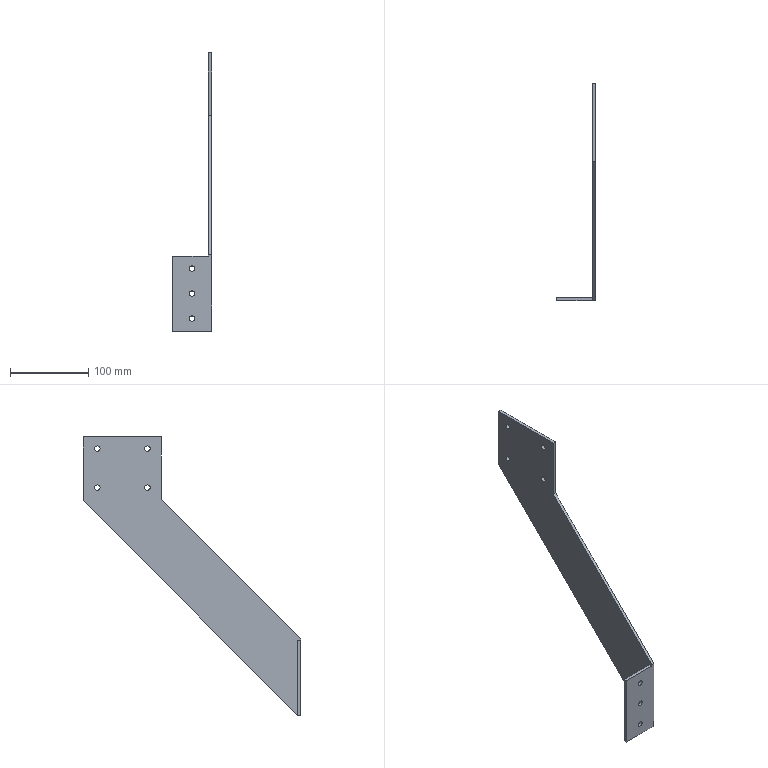Component | SolidWorks | BeltLineSupportPlate-1 | 1 solid | 26 faces | box 50 x 278.18 x 356 mm | volume 141854 mm3 | cylinder 14 | plane 12 | commonest cylinder face diameters 7 x14
STEP:
#1=COLOUR_RGB('',0.7922,0.8196,0.9333);
#2=FILL_AREA_STYLE_COLOUR('',#1);
#3=FILL_AREA_STYLE('',(#2));
#4=SURFACE_STYLE_FILL_AREA(#3);
#5=SURFACE_SIDE_STYLE('',(#4));
#6=SURFACE_STYLE_USAGE(.BOTH.,#5);
#7=PRESENTATION_STYLE_ASSIGNMENT((#6));
#8=CARTESIAN_POINT('',(239.429,105.032,-7.426));
#9=VERTEX_POINT('',#8);
#10=CARTESIAN_POINT('',(239.154,105.032,-7.426));
#11=VERTEX_POINT('',#10);
#12=CARTESIAN_POINT('',(239.292,105.032,-7.426));
#13=DIRECTION('',(0.,-1.,-0.));
#14=DIRECTION('',(0.,0.,1.));
#15=AXIS2_PLACEMENT_3D('',#12,#13,#14);
#16=CIRCLE('',#15,0.1378);
#17=EDGE_CURVE('',#9,#11,#16,.T.);
#18=ORIENTED_EDGE('',*,*,#17,.T.);
#19=CARTESIAN_POINT('',(239.154,105.19,-7.426));
#20=VERTEX_POINT('',#19);
#21=CARTESIAN_POINT('',(239.154,105.19,-7.426));
#22=DIRECTION('',(-0.,1.,0.));
#23=VECTOR('',#22,39.37);
#24=LINE('',#21,#23);
#25=EDGE_CURVE('',#11,#20,#24,.T.);
#26=ORIENTED_EDGE('',*,*,#25,.T.);
#27=CARTESIAN_POINT('',(239.429,105.19,-7.426));
#28=VERTEX_POINT('',#27);
#29=CARTESIAN_POINT('',(239.292,105.19,-7.426));
#30=DIRECTION('',(-0.,1.,0.));
#31=DIRECTION('',(1.,0.,0.));
#32=AXIS2_PLACEMENT_3D('',#29,#30,#31);
#33=CIRCLE('',#32,0.1378);
#34=EDGE_CURVE('',#20,#28,#33,.T.);
#35=ORIENTED_EDGE('',*,*,#34,.T.);
#36=CARTESIAN_POINT('',(239.429,105.19,-7.426));
#37=DIRECTION('',(-0.,1.,0.));
#38=VECTOR('',#37,39.37);
#39=LINE('',#36,#38);
#40=EDGE_CURVE('',#9,#28,#39,.T.);
#41=ORIENTED_EDGE('',*,*,#40,.F.);
#42=EDGE_LOOP('',(#18,#26,#35,#41));
#43=FACE_OUTER_BOUND('',#42,.T.);
#44=CARTESIAN_POINT('',(239.292,105.19,-7.426));
#45=DIRECTION('',(-0.,1.,0.));
#46=DIRECTION('',(1.,0.,0.));
#47=AXIS2_PLACEMENT_3D('',#44,#45,#46);
#48=CYLINDRICAL_SURFACE('',#47,0.1378);
#49=ADVANCED_FACE('',(#43),#48,.F.);
#50=CARTESIAN_POINT('',(239.429,105.032,-8.686));
#51=VERTEX_POINT('',#50);
#52=CARTESIAN_POINT('',(239.154,105.032,-8.686));
#53=VERTEX_POINT('',#52);
#54=CARTESIAN_POINT('',(239.292,105.032,-8.686));
#55=DIRECTION('',(0.,-1.,-0.));
#56=DIRECTION('',(0.,0.,1.));
#57=AXIS2_PLACEMENT_3D('',#54,#55,#56);
#58=CIRCLE('',#57,0.1378);
#59=EDGE_CURVE('',#51,#53,#58,.T.);
#60=ORIENTED_EDGE('',*,*,#59,.T.);
#61=CARTESIAN_POINT('',(239.154,105.19,-8.686));
#62=VERTEX_POINT('',#61);
#63=CARTESIAN_POINT('',(239.154,105.19,-8.686));
#64=DIRECTION('',(-0.,1.,0.));
#65=VECTOR('',#64,39.37);
#66=LINE('',#63,#65);
#67=EDGE_CURVE('',#53,#62,#66,.T.);
#68=ORIENTED_EDGE('',*,*,#67,.T.);
#69=CARTESIAN_POINT('',(239.429,105.19,-8.686));
#70=VERTEX_POINT('',#69);
#71=CARTESIAN_POINT('',(239.292,105.19,-8.686));
#72=DIRECTION('',(-0.,1.,0.));
#73=DIRECTION('',(1.,0.,0.));
#74=AXIS2_PLACEMENT_3D('',#71,#72,#73);
#75=CIRCLE('',#74,0.1378);
#76=EDGE_CURVE('',#62,#70,#75,.T.);
#77=ORIENTED_EDGE('',*,*,#76,.T.);
#78=CARTESIAN_POINT('',(239.429,105.19,-8.686));
#79=DIRECTION('',(-0.,1.,0.));
#80=VECTOR('',#79,39.37);
#81=LINE('',#78,#80);
#82=EDGE_CURVE('',#51,#70,#81,.T.);
#83=ORIENTED_EDGE('',*,*,#82,.F.);
#84=EDGE_LOOP('',(#60,#68,#77,#83));
#85=FACE_OUTER_BOUND('',#84,.T.);
#86=CARTESIAN_POINT('',(239.292,105.19,-8.686));
#87=DIRECTION('',(-0.,1.,0.));
#88=DIRECTION('',(1.,0.,0.));
#89=AXIS2_PLACEMENT_3D('',#86,#87,#88);
#90=CYLINDRICAL_SURFACE('',#89,0.1378);
#91=ADVANCED_FACE('',(#85),#90,.F.);
#92=CARTESIAN_POINT('',(239.429,105.032,-9.946));
#93=VERTEX_POINT('',#92);
#94=CARTESIAN_POINT('',(239.154,105.032,-9.946));
#95=VERTEX_POINT('',#94);
#96=CARTESIAN_POINT('',(239.292,105.032,-9.946));
#97=DIRECTION('',(0.,-1.,-0.));
#98=DIRECTION('',(0.,0.,1.));
#99=AXIS2_PLACEMENT_3D('',#96,#97,#98);
#100=CIRCLE('',#99,0.1378);
#101=EDGE_CURVE('',#93,#95,#100,.T.);
#102=ORIENTED_EDGE('',*,*,#101,.T.);
#103=CARTESIAN_POINT('',(239.154,105.19,-9.946));
#104=VERTEX_POINT('',#103);
#105=CARTESIAN_POINT('',(239.154,105.19,-9.946));
#106=DIRECTION('',(-0.,1.,0.));
#107=VECTOR('',#106,39.37);
#108=LINE('',#105,#107);
#109=EDGE_CURVE('',#95,#104,#108,.T.);
#110=ORIENTED_EDGE('',*,*,#109,.T.);
#111=CARTESIAN_POINT('',(239.429,105.19,-9.946));
#112=VERTEX_POINT('',#111);
#113=CARTESIAN_POINT('',(239.292,105.19,-9.946));
#114=DIRECTION('',(-0.,1.,0.));
#115=DIRECTION('',(1.,0.,0.));
#116=AXIS2_PLACEMENT_3D('',#113,#114,#115);
#117=CIRCLE('',#116,0.1378);
#118=EDGE_CURVE('',#104,#112,#117,.T.);
#119=ORIENTED_EDGE('',*,*,#118,.T.);
#120=CARTESIAN_POINT('',(239.429,105.19,-9.946));
#121=DIRECTION('',(-0.,1.,0.));
#122=VECTOR('',#121,39.37);
#123=LINE('',#120,#122);
#124=EDGE_CURVE('',#93,#112,#123,.T.);
#125=ORIENTED_EDGE('',*,*,#124,.F.);
#126=EDGE_LOOP('',(#102,#110,#119,#125));
#127=FACE_OUTER_BOUND('',#126,.T.);
#128=CARTESIAN_POINT('',(239.292,105.19,-9.946));
#129=DIRECTION('',(-0.,1.,0.));
#130=DIRECTION('',(1.,0.,0.));
#131=AXIS2_PLACEMENT_3D('',#128,#129,#130);
#132=CYLINDRICAL_SURFACE('',#131,0.1378);
#133=ADVANCED_FACE('',(#127),#132,.F.);
#134=CARTESIAN_POINT('',(240.276,112.618,0.8809));
#135=VERTEX_POINT('',#134);
#136=CARTESIAN_POINT('',(240.276,112.894,0.8809));
#137=VERTEX_POINT('',#136);
#138=CARTESIAN_POINT('',(240.276,112.756,0.8809));
#139=DIRECTION('',(-1.,-0.,-0.));
#140=DIRECTION('',(0.,1.,0.));
#141=AXIS2_PLACEMENT_3D('',#138,#139,#140);
#142=CIRCLE('',#141,0.1378);
#143=EDGE_CURVE('',#135,#137,#142,.T.);
#144=ORIENTED_EDGE('',*,*,#143,.F.);
#145=CARTESIAN_POINT('',(240.118,112.618,0.8809));
#146=VERTEX_POINT('',#145);
#147=CARTESIAN_POINT('',(240.118,112.618,0.8809));
#148=DIRECTION('',(-1.,-0.,-0.));
#149=VECTOR('',#148,39.37);
#150=LINE('',#147,#149);
#151=EDGE_CURVE('',#135,#146,#150,.T.);
#152=ORIENTED_EDGE('',*,*,#151,.T.);
#153=CARTESIAN_POINT('',(240.118,112.894,0.8809));
#154=VERTEX_POINT('',#153);
#155=CARTESIAN_POINT('',(240.118,112.756,0.8809));
#156=DIRECTION('',(-1.,-0.,-0.));
#157=DIRECTION('',(0.,1.,0.));
#158=AXIS2_PLACEMENT_3D('',#155,#156,#157);
#159=CIRCLE('',#158,0.1378);
#160=EDGE_CURVE('',#146,#154,#159,.T.);
#161=ORIENTED_EDGE('',*,*,#160,.T.);
#162=CARTESIAN_POINT('',(240.118,112.894,0.8809));
#163=DIRECTION('',(-1.,-0.,-0.));
#164=VECTOR('',#163,39.37);
#165=LINE('',#162,#164);
#166=EDGE_CURVE('',#137,#154,#165,.T.);
#167=ORIENTED_EDGE('',*,*,#166,.F.);
#168=EDGE_LOOP('',(#144,#152,#161,#167));
#169=FACE_OUTER_BOUND('',#168,.T.);
#170=CARTESIAN_POINT('',(240.118,112.756,0.8809));
#171=DIRECTION('',(-1.,-0.,-0.));
#172=DIRECTION('',(0.,1.,0.));
#173=AXIS2_PLACEMENT_3D('',#170,#171,#172);
#174=CYLINDRICAL_SURFACE('',#173,0.1378);
#175=ADVANCED_FACE('',(#169),#174,.F.);
#176=CARTESIAN_POINT('',(240.276,115.138,0.8809));
#177=VERTEX_POINT('',#176);
#178=CARTESIAN_POINT('',(240.276,115.413,0.8809));
#179=VERTEX_POINT('',#178);
#180=CARTESIAN_POINT('',(240.276,115.275,0.8809));
#181=DIRECTION('',(-1.,-0.,-0.));
#182=DIRECTION('',(0.,1.,0.));
#183=AXIS2_PLACEMENT_3D('',#180,#181,#182);
#184=CIRCLE('',#183,0.1378);
#185=EDGE_CURVE('',#177,#179,#184,.T.);
#186=ORIENTED_EDGE('',*,*,#185,.F.);
#187=CARTESIAN_POINT('',(240.118,115.138,0.8809));
#188=VERTEX_POINT('',#187);
#189=CARTESIAN_POINT('',(240.118,115.138,0.8809));
#190=DIRECTION('',(-1.,-0.,-0.));
#191=VECTOR('',#190,39.37);
#192=LINE('',#189,#191);
#193=EDGE_CURVE('',#177,#188,#192,.T.);
#194=ORIENTED_EDGE('',*,*,#193,.T.);
#195=CARTESIAN_POINT('',(240.118,115.413,0.8809));
#196=VERTEX_POINT('',#195);
#197=CARTESIAN_POINT('',(240.118,115.275,0.8809));
#198=DIRECTION('',(-1.,-0.,-0.));
#199=DIRECTION('',(0.,1.,0.));
#200=AXIS2_PLACEMENT_3D('',#197,#198,#199);
#201=CIRCLE('',#200,0.1378);
#202=EDGE_CURVE('',#188,#196,#201,.T.);
#203=ORIENTED_EDGE('',*,*,#202,.T.);
#204=CARTESIAN_POINT('',(240.118,115.413,0.8809));
#205=DIRECTION('',(-1.,-0.,-0.));
#206=VECTOR('',#205,39.37);
#207=LINE('',#204,#206);
#208=EDGE_CURVE('',#179,#196,#207,.T.);
#209=ORIENTED_EDGE('',*,*,#208,.F.);
#210=EDGE_LOOP('',(#186,#194,#203,#209));
#211=FACE_OUTER_BOUND('',#210,.T.);
#212=CARTESIAN_POINT('',(240.118,115.275,0.8809));
#213=DIRECTION('',(-1.,-0.,-0.));
#214=DIRECTION('',(0.,1.,0.));
#215=AXIS2_PLACEMENT_3D('',#212,#213,#214);
#216=CYLINDRICAL_SURFACE('',#215,0.1378);
#217=ADVANCED_FACE('',(#211),#216,.F.);
#218=CARTESIAN_POINT('',(240.276,115.138,2.849));
#219=VERTEX_POINT('',#218);
#220=CARTESIAN_POINT('',(240.276,115.413,2.849));
#221=VERTEX_POINT('',#220);
#222=CARTESIAN_POINT('',(240.276,115.275,2.849));
#223=DIRECTION('',(-1.,-0.,-0.));
#224=DIRECTION('',(0.,1.,0.));
#225=AXIS2_PLACEMENT_3D('',#222,#223,#224);
#226=CIRCLE('',#225,0.1378);
#227=EDGE_CURVE('',#219,#221,#226,.T.);
#228=ORIENTED_EDGE('',*,*,#227,.F.);
#229=CARTESIAN_POINT('',(240.118,115.138,2.849));
#230=VERTEX_POINT('',#229);
#231=CARTESIAN_POINT('',(240.118,115.138,2.849));
#232=DIRECTION('',(-1.,-0.,-0.));
#233=VECTOR('',#232,39.37);
#234=LINE('',#231,#233);
#235=EDGE_CURVE('',#219,#230,#234,.T.);
#236=ORIENTED_EDGE('',*,*,#235,.T.);
#237=CARTESIAN_POINT('',(240.118,115.413,2.849));
#238=VERTEX_POINT('',#237);
#239=CARTESIAN_POINT('',(240.118,115.275,2.849));
#240=DIRECTION('',(-1.,-0.,-0.));
#241=DIRECTION('',(0.,1.,0.));
#242=AXIS2_PLACEMENT_3D('',#239,#240,#241);
#243=CIRCLE('',#242,0.1378);
#244=EDGE_CURVE('',#230,#238,#243,.T.);
#245=ORIENTED_EDGE('',*,*,#244,.T.);
#246=CARTESIAN_POINT('',(240.118,115.413,2.849));
#247=DIRECTION('',(-1.,-0.,-0.));
#248=VECTOR('',#247,39.37);
#249=LINE('',#246,#248);
#250=EDGE_CURVE('',#221,#238,#249,.T.);
#251=ORIENTED_EDGE('',*,*,#250,.F.);
#252=EDGE_LOOP('',(#228,#236,#245,#251));
#253=FACE_OUTER_BOUND('',#252,.T.);
#254=CARTESIAN_POINT('',(240.118,115.275,2.849));
#255=DIRECTION('',(-1.,-0.,-0.));
#256=DIRECTION('',(0.,1.,0.));
#257=AXIS2_PLACEMENT_3D('',#254,#255,#256);
#258=CYLINDRICAL_SURFACE('',#257,0.1378);
#259=ADVANCED_FACE('',(#253),#258,.F.);
#260=CARTESIAN_POINT('',(240.276,112.618,2.849));
#261=VERTEX_POINT('',#260);
#262=CARTESIAN_POINT('',(240.276,112.894,2.849));
#263=VERTEX_POINT('',#262);
#264=CARTESIAN_POINT('',(240.276,112.756,2.849));
#265=DIRECTION('',(-1.,-0.,-0.));
#266=DIRECTION('',(0.,1.,0.));
#267=AXIS2_PLACEMENT_3D('',#264,#265,#266);
#268=CIRCLE('',#267,0.1378);
#269=EDGE_CURVE('',#261,#263,#268,.T.);
#270=ORIENTED_EDGE('',*,*,#269,.F.);
#271=CARTESIAN_POINT('',(240.118,112.618,2.849));
#272=VERTEX_POINT('',#271);
#273=CARTESIAN_POINT('',(240.118,112.618,2.849));
#274=DIRECTION('',(-1.,-0.,-0.));
#275=VECTOR('',#274,39.37);
#276=LINE('',#273,#275);
#277=EDGE_CURVE('',#261,#272,#276,.T.);
#278=ORIENTED_EDGE('',*,*,#277,.T.);
#279=CARTESIAN_POINT('',(240.118,112.894,2.849));
#280=VERTEX_POINT('',#279);
#281=CARTESIAN_POINT('',(240.118,112.756,2.849));
#282=DIRECTION('',(-1.,-0.,-0.));
#283=DIRECTION('',(0.,1.,0.));
#284=AXIS2_PLACEMENT_3D('',#281,#282,#283);
#285=CIRCLE('',#284,0.1378);
#286=EDGE_CURVE('',#272,#280,#285,.T.);
#287=ORIENTED_EDGE('',*,*,#286,.T.);
#288=CARTESIAN_POINT('',(240.118,112.894,2.849));
#289=DIRECTION('',(-1.,-0.,-0.));
#290=VECTOR('',#289,39.37);
#291=LINE('',#288,#290);
#292=EDGE_CURVE('',#263,#280,#291,.T.);
#293=ORIENTED_EDGE('',*,*,#292,.F.);
#294=EDGE_LOOP('',(#270,#278,#287,#293));
#295=FACE_OUTER_BOUND('',#294,.T.);
#296=CARTESIAN_POINT('',(240.118,112.756,2.849));
#297=DIRECTION('',(-1.,-0.,-0.));
#298=DIRECTION('',(0.,1.,0.));
#299=AXIS2_PLACEMENT_3D('',#296,#297,#298);
#300=CYLINDRICAL_SURFACE('',#299,0.1378);
#301=ADVANCED_FACE('',(#295),#300,.F.);
#302=CARTESIAN_POINT('',(240.276,105.19,-10.576));
#303=VERTEX_POINT('',#302);
#304=CARTESIAN_POINT('',(240.276,105.032,-10.576));
#305=VERTEX_POINT('',#304);
#306=CARTESIAN_POINT('',(240.276,103.386,-10.576));
#307=DIRECTION('',(0.,-1.,-0.));
#308=VECTOR('',#307,39.37);
#309=LINE('',#306,#308);
#310=EDGE_CURVE('',#303,#305,#309,.T.);
#311=ORIENTED_EDGE('',*,*,#310,.T.);
#312=CARTESIAN_POINT('',(238.307,105.032,-10.576));
#313=VERTEX_POINT('',#312);
#314=CARTESIAN_POINT('',(238.307,105.032,-10.576));
#315=DIRECTION('',(1.,0.,0.));
#316=VECTOR('',#315,39.37);
#317=LINE('',#314,#316);
#318=EDGE_CURVE('',#313,#305,#317,.T.);
#319=ORIENTED_EDGE('',*,*,#318,.F.);
#320=CARTESIAN_POINT('',(238.307,105.19,-10.576));
#321=VERTEX_POINT('',#320);
#322=CARTESIAN_POINT('',(238.307,105.19,-10.576));
#323=DIRECTION('',(-0.,1.,0.));
#324=VECTOR('',#323,39.37);
#325=LINE('',#322,#324);
#326=EDGE_CURVE('',#313,#321,#325,.T.);
#327=ORIENTED_EDGE('',*,*,#326,.T.);
#328=CARTESIAN_POINT('',(240.118,105.19,-10.576));
#329=VERTEX_POINT('',#328);
#330=CARTESIAN_POINT('',(238.307,105.19,-10.576));
#331=DIRECTION('',(1.,0.,0.));
#332=VECTOR('',#331,39.37);
#333=LINE('',#330,#332);
#334=EDGE_CURVE('',#321,#329,#333,.T.);
#335=ORIENTED_EDGE('',*,*,#334,.T.);
#336=CARTESIAN_POINT('',(240.118,105.19,-10.576));
#337=DIRECTION('',(1.,0.,0.));
#338=VECTOR('',#337,39.37);
#339=LINE('',#336,#338);
#340=EDGE_CURVE('',#329,#303,#339,.T.);
#341=ORIENTED_EDGE('',*,*,#340,.T.);
#342=EDGE_LOOP('',(#311,#319,#327,#335,#341));
#343=FACE_OUTER_BOUND('',#342,.T.);
#344=CARTESIAN_POINT('',(240.118,103.386,-10.576));
#345=DIRECTION('',(-0.,-0.,1.));
#346=DIRECTION('',(1.,0.,0.));
#347=AXIS2_PLACEMENT_3D('',#344,#345,#346);
#348=PLANE('',#347);
#349=ADVANCED_FACE('',(#343),#348,.F.);
#350=CARTESIAN_POINT('',(240.118,105.032,-6.724));
#351=VERTEX_POINT('',#350);
#352=CARTESIAN_POINT('',(240.118,112.047,0.2904));
#353=VERTEX_POINT('',#352);
#354=CARTESIAN_POINT('',(240.118,112.047,0.2904));
#355=DIRECTION('',(-0.,0.7071,0.7071));
#356=VECTOR('',#355,39.37);
#357=LINE('',#354,#356);
#358=EDGE_CURVE('',#351,#353,#357,.T.);
#359=ORIENTED_EDGE('',*,*,#358,.F.);
#360=CARTESIAN_POINT('',(240.276,105.032,-6.724));
#361=VERTEX_POINT('',#360);
#362=CARTESIAN_POINT('',(242.087,105.032,-6.724));
#363=DIRECTION('',(-1.,-0.,-0.));
#364=VECTOR('',#363,39.37);
#365=LINE('',#362,#364);
#366=EDGE_CURVE('',#361,#351,#365,.T.);
#367=ORIENTED_EDGE('',*,*,#366,.F.);
#368=CARTESIAN_POINT('',(240.276,112.047,0.2904));
#369=VERTEX_POINT('',#368);
#370=CARTESIAN_POINT('',(240.276,112.047,0.2904));
#371=DIRECTION('',(-0.,0.7071,0.7071));
#372=VECTOR('',#371,39.37);
#373=LINE('',#370,#372);
#374=EDGE_CURVE('',#361,#369,#373,.T.);
#375=ORIENTED_EDGE('',*,*,#374,.T.);
#376=CARTESIAN_POINT('',(240.118,112.047,0.2904));
#377=DIRECTION('',(1.,0.,0.));
#378=VECTOR('',#377,39.37);
#379=LINE('',#376,#378);
#380=EDGE_CURVE('',#353,#369,#379,.T.);
#381=ORIENTED_EDGE('',*,*,#380,.F.);
#382=EDGE_LOOP('',(#359,#367,#375,#381));
#383=FACE_OUTER_BOUND('',#382,.T.);
#384=CARTESIAN_POINT('',(240.118,112.047,0.2904));
#385=DIRECTION('',(-0.,0.7071,-0.7071));
#386=DIRECTION('',(0.,-0.7071,-0.7071));
#387=AXIS2_PLACEMENT_3D('',#384,#385,#386);
#388=PLANE('',#387);
#389=ADVANCED_FACE('',(#383),#388,.F.);
#390=CARTESIAN_POINT('',(240.276,112.047,3.44));
#391=VERTEX_POINT('',#390);
#392=CARTESIAN_POINT('',(240.276,112.047,3.44));
#393=DIRECTION('',(-0.,0.,1.));
#394=VECTOR('',#393,39.37);
#395=LINE('',#392,#394);
#396=EDGE_CURVE('',#369,#391,#395,.T.);
#397=ORIENTED_EDGE('',*,*,#396,.T.);
#398=CARTESIAN_POINT('',(240.118,112.047,3.44));
#399=VERTEX_POINT('',#398);
#400=CARTESIAN_POINT('',(240.118,112.047,3.44));
#401=DIRECTION('',(1.,0.,0.));
#402=VECTOR('',#401,39.37);
#403=LINE('',#400,#402);
#404=EDGE_CURVE('',#399,#391,#403,.T.);
#405=ORIENTED_EDGE('',*,*,#404,.F.);
#406=CARTESIAN_POINT('',(240.118,112.047,3.44));
#407=DIRECTION('',(-0.,0.,1.));
#408=VECTOR('',#407,39.37);
#409=LINE('',#406,#408);
#410=EDGE_CURVE('',#353,#399,#409,.T.);
#411=ORIENTED_EDGE('',*,*,#410,.F.);
#412=ORIENTED_EDGE('',*,*,#380,.T.);
#413=EDGE_LOOP('',(#397,#405,#411,#412));
#414=FACE_OUTER_BOUND('',#413,.T.);
#415=CARTESIAN_POINT('',(240.118,112.047,3.44));
#416=DIRECTION('',(-0.,1.,-0.));
#417=DIRECTION('',(0.,-0.,-1.));
#418=AXIS2_PLACEMENT_3D('',#415,#416,#417);
#419=PLANE('',#418);
#420=ADVANCED_FACE('',(#414),#419,.F.);
#421=CARTESIAN_POINT('',(240.276,115.984,3.44));
#422=VERTEX_POINT('',#421);
#423=CARTESIAN_POINT('',(240.276,115.984,3.44));
#424=DIRECTION('',(-0.,1.,0.));
#425=VECTOR('',#424,39.37);
#426=LINE('',#423,#425);
#427=EDGE_CURVE('',#391,#422,#426,.T.);
#428=ORIENTED_EDGE('',*,*,#427,.T.);
#429=CARTESIAN_POINT('',(240.118,115.984,3.44));
#430=VERTEX_POINT('',#429);
#431=CARTESIAN_POINT('',(240.118,115.984,3.44));
#432=DIRECTION('',(1.,0.,0.));
#433=VECTOR('',#432,39.37);
#434=LINE('',#431,#433);
#435=EDGE_CURVE('',#430,#422,#434,.T.);
#436=ORIENTED_EDGE('',*,*,#435,.F.);
#437=CARTESIAN_POINT('',(240.118,115.984,3.44));
#438=DIRECTION('',(-0.,1.,0.));
#439=VECTOR('',#438,39.37);
#440=LINE('',#437,#439);
#441=EDGE_CURVE('',#399,#430,#440,.T.);
#442=ORIENTED_EDGE('',*,*,#441,.F.);
#443=ORIENTED_EDGE('',*,*,#404,.T.);
#444=EDGE_LOOP('',(#428,#436,#442,#443));
#445=FACE_OUTER_BOUND('',#444,.T.);
#446=CARTESIAN_POINT('',(240.118,115.984,3.44));
#447=DIRECTION('',(0.,0.,-1.));
#448=DIRECTION('',(0.,-1.,-0.));
#449=AXIS2_PLACEMENT_3D('',#446,#447,#448);
#450=PLANE('',#449);
#451=ADVANCED_FACE('',(#445),#450,.F.);
#452=CARTESIAN_POINT('',(240.276,115.984,0.2186));
#453=VERTEX_POINT('',#452);
#454=CARTESIAN_POINT('',(240.276,115.984,0.2186));
#455=DIRECTION('',(0.,0.,-1.));
#456=VECTOR('',#455,39.37);
#457=LINE('',#454,#456);
#458=EDGE_CURVE('',#422,#453,#457,.T.);
#459=ORIENTED_EDGE('',*,*,#458,.T.);
#460=CARTESIAN_POINT('',(240.118,115.984,0.2186));
#461=VERTEX_POINT('',#460);
#462=CARTESIAN_POINT('',(240.118,115.984,0.2186));
#463=DIRECTION('',(1.,0.,0.));
#464=VECTOR('',#463,39.37);
#465=LINE('',#462,#464);
#466=EDGE_CURVE('',#461,#453,#465,.T.);
#467=ORIENTED_EDGE('',*,*,#466,.F.);
#468=CARTESIAN_POINT('',(240.118,115.984,0.2186));
#469=DIRECTION('',(0.,0.,-1.));
#470=VECTOR('',#469,39.37);
#471=LINE('',#468,#470);
#472=EDGE_CURVE('',#430,#461,#471,.T.);
#473=ORIENTED_EDGE('',*,*,#472,.F.);
#474=ORIENTED_EDGE('',*,*,#435,.T.);
#475=EDGE_LOOP('',(#459,#467,#473,#474));
#476=FACE_OUTER_BOUND('',#475,.T.);
#477=CARTESIAN_POINT('',(240.118,115.984,0.2186));
#478=DIRECTION('',(0.,-1.,-0.));
#479=DIRECTION('',(-1.,-0.,-0.));
#480=AXIS2_PLACEMENT_3D('',#477,#478,#479);
#481=PLANE('',#480);
#482=ADVANCED_FACE('',(#476),#481,.F.);
#483=CARTESIAN_POINT('',(240.276,105.19,-10.576));
#484=DIRECTION('',(0.,-0.7071,-0.7071));
#485=VECTOR('',#484,39.37);
#486=LINE('',#483,#485);
#487=EDGE_CURVE('',#453,#303,#486,.T.);
#488=ORIENTED_EDGE('',*,*,#487,.T.);
#489=ORIENTED_EDGE('',*,*,#340,.F.);
#490=CARTESIAN_POINT('',(240.118,105.19,-10.576));
#491=DIRECTION('',(0.,-0.7071,-0.7071));
#492=VECTOR('',#491,39.37);
#493=LINE('',#490,#492);
#494=EDGE_CURVE('',#461,#329,#493,.T.);
#495=ORIENTED_EDGE('',*,*,#494,.F.);
#496=ORIENTED_EDGE('',*,*,#466,.T.);
#497=EDGE_LOOP('',(#488,#489,#495,#496));
#498=FACE_OUTER_BOUND('',#497,.T.);
#499=CARTESIAN_POINT('',(240.118,105.19,-10.576));
#500=DIRECTION('',(0.,-0.7071,0.7071));
#501=DIRECTION('',(-0.,0.7071,0.7071));
#502=AXIS2_PLACEMENT_3D('',#499,#500,#501);
#503=PLANE('',#502);
#504=ADVANCED_FACE('',(#498),#503,.F.);
#505=CARTESIAN_POINT('',(240.118,112.756,0.8809));
#506=DIRECTION('',(-1.,-0.,-0.));
#507=DIRECTION('',(0.,1.,0.));
#508=AXIS2_PLACEMENT_3D('',#505,#506,#507);
#509=CIRCLE('',#508,0.1378);
#510=EDGE_CURVE('',#154,#146,#509,.T.);
#511=ORIENTED_EDGE('',*,*,#510,.F.);
#512=ORIENTED_EDGE('',*,*,#160,.F.);
#513=EDGE_LOOP('',(#511,#512));
#514=FACE_BOUND('',#513,.T.);
#515=CARTESIAN_POINT('',(240.118,115.275,0.8809));
#516=DIRECTION('',(-1.,-0.,-0.));
#517=DIRECTION('',(0.,1.,0.));
#518=AXIS2_PLACEMENT_3D('',#515,#516,#517);
#519=CIRCLE('',#518,0.1378);
#520=EDGE_CURVE('',#196,#188,#519,.T.);
#521=ORIENTED_EDGE('',*,*,#520,.F.);
#522=ORIENTED_EDGE('',*,*,#202,.F.);
#523=EDGE_LOOP('',(#521,#522));
#524=FACE_BOUND('',#523,.T.);
#525=CARTESIAN_POINT('',(240.118,115.275,2.849));
#526=DIRECTION('',(-1.,-0.,-0.));
#527=DIRECTION('',(0.,1.,0.));
#528=AXIS2_PLACEMENT_3D('',#525,#526,#527);
#529=CIRCLE('',#528,0.1378);
#530=EDGE_CURVE('',#238,#230,#529,.T.);
#531=ORIENTED_EDGE('',*,*,#530,.F.);
#532=ORIENTED_EDGE('',*,*,#244,.F.);
#533=EDGE_LOOP('',(#531,#532));
#534=FACE_BOUND('',#533,.T.);
#535=CARTESIAN_POINT('',(240.118,112.756,2.849));
#536=DIRECTION('',(-1.,-0.,-0.));
#537=DIRECTION('',(0.,1.,0.));
#538=AXIS2_PLACEMENT_3D('',#535,#536,#537);
#539=CIRCLE('',#538,0.1378);
#540=EDGE_CURVE('',#280,#272,#539,.T.);
#541=ORIENTED_EDGE('',*,*,#540,.F.);
#542=ORIENTED_EDGE('',*,*,#286,.F.);
#543=EDGE_LOOP('',(#541,#542));
#544=FACE_BOUND('',#543,.T.);
#545=CARTESIAN_POINT('',(240.118,105.19,-6.796));
#546=VERTEX_POINT('',#545);
#547=CARTESIAN_POINT('',(240.118,105.032,-6.796));
#548=VERTEX_POINT('',#547);
#549=CARTESIAN_POINT('',(240.118,103.386,-6.796));
#550=DIRECTION('',(0.,-1.,-0.));
#551=VECTOR('',#550,39.37);
#552=LINE('',#549,#551);
#553=EDGE_CURVE('',#546,#548,#552,.T.);
#554=ORIENTED_EDGE('',*,*,#553,.T.);
#555=CARTESIAN_POINT('',(240.118,105.032,-10.576));
#556=DIRECTION('',(0.,0.,-1.));
#557=VECTOR('',#556,39.37);
#558=LINE('',#555,#557);
#559=EDGE_CURVE('',#351,#548,#558,.T.);
#560=ORIENTED_EDGE('',*,*,#559,.F.);
#561=ORIENTED_EDGE('',*,*,#358,.T.);
#562=ORIENTED_EDGE('',*,*,#410,.T.);
#563=ORIENTED_EDGE('',*,*,#441,.T.);
#564=ORIENTED_EDGE('',*,*,#472,.T.);
#565=ORIENTED_EDGE('',*,*,#494,.T.);
#566=CARTESIAN_POINT('',(240.118,105.19,-10.576));
#567=DIRECTION('',(-0.,-0.,1.));
#568=VECTOR('',#567,39.37);
#569=LINE('',#566,#568);
#570=EDGE_CURVE('',#329,#546,#569,.T.);
#571=ORIENTED_EDGE('',*,*,#570,.T.);
#572=EDGE_LOOP('',(#554,#560,#561,#562,#563,#564,#565,#571));
#573=FACE_OUTER_BOUND('',#572,.T.);
#574=CARTESIAN_POINT('',(240.118,103.386,-10.576));
#575=DIRECTION('',(1.,0.,0.));
#576=DIRECTION('',(0.,-1.,-0.));
#577=AXIS2_PLACEMENT_3D('',#574,#575,#576);
#578=PLANE('',#577);
#579=ADVANCED_FACE('',(#514,#524,#534,#544,#573),#578,.F.);
#580=CARTESIAN_POINT('',(240.276,105.032,-10.576));
#581=DIRECTION('',(-0.,-0.,1.));
#582=VECTOR('',#581,39.37);
#583=LINE('',#580,#582);
#584=EDGE_CURVE('',#305,#361,#583,.T.);
#585=ORIENTED_EDGE('',*,*,#584,.F.);
#586=ORIENTED_EDGE('',*,*,#310,.F.);
#587=ORIENTED_EDGE('',*,*,#487,.F.);
#588=ORIENTED_EDGE('',*,*,#458,.F.);
#589=ORIENTED_EDGE('',*,*,#427,.F.);
#590=ORIENTED_EDGE('',*,*,#396,.F.);
#591=ORIENTED_EDGE('',*,*,#374,.F.);
#592=EDGE_LOOP('',(#585,#586,#587,#588,#589,#590,#591));
#593=FACE_OUTER_BOUND('',#592,.T.);
#594=CARTESIAN_POINT('',(240.276,112.756,0.8809));
#595=DIRECTION('',(-1.,-0.,-0.));
#596=DIRECTION('',(0.,1.,0.));
#597=AXIS2_PLACEMENT_3D('',#594,#595,#596);
#598=CIRCLE('',#597,0.1378);
#599=EDGE_CURVE('',#137,#135,#598,.T.);
#600=ORIENTED_EDGE('',*,*,#599,.T.);
#601=ORIENTED_EDGE('',*,*,#143,.T.);
#602=EDGE_LOOP('',(#600,#601));
#603=FACE_BOUND('',#602,.T.);
#604=CARTESIAN_POINT('',(240.276,115.275,0.8809));
#605=DIRECTION('',(-1.,-0.,-0.));
#606=DIRECTION('',(0.,1.,0.));
#607=AXIS2_PLACEMENT_3D('',#604,#605,#606);
#608=CIRCLE('',#607,0.1378);
#609=EDGE_CURVE('',#179,#177,#608,.T.);
#610=ORIENTED_EDGE('',*,*,#609,.T.);
#611=ORIENTED_EDGE('',*,*,#185,.T.);
#612=EDGE_LOOP('',(#610,#611));
#613=FACE_BOUND('',#612,.T.);
#614=CARTESIAN_POINT('',(240.276,115.275,2.849));
#615=DIRECTION('',(-1.,-0.,-0.));
#616=DIRECTION('',(0.,1.,0.));
#617=AXIS2_PLACEMENT_3D('',#614,#615,#616);
#618=CIRCLE('',#617,0.1378);
#619=EDGE_CURVE('',#221,#219,#618,.T.);
#620=ORIENTED_EDGE('',*,*,#619,.T.);
#621=ORIENTED_EDGE('',*,*,#227,.T.);
#622=EDGE_LOOP('',(#620,#621));
#623=FACE_BOUND('',#622,.T.);
#624=CARTESIAN_POINT('',(240.276,112.756,2.849));
#625=DIRECTION('',(-1.,-0.,-0.));
#626=DIRECTION('',(0.,1.,0.));
#627=AXIS2_PLACEMENT_3D('',#624,#625,#626);
#628=CIRCLE('',#627,0.1378);
#629=EDGE_CURVE('',#263,#261,#628,.T.);
#630=ORIENTED_EDGE('',*,*,#629,.T.);
#631=ORIENTED_EDGE('',*,*,#269,.T.);
#632=EDGE_LOOP('',(#630,#631));
#633=FACE_BOUND('',#632,.T.);
#634=CARTESIAN_POINT('',(240.276,103.386,-10.576));
#635=DIRECTION('',(1.,0.,0.));
#636=DIRECTION('',(0.,-1.,-0.));
#637=AXIS2_PLACEMENT_3D('',#634,#635,#636);
#638=PLANE('',#637);
#639=ADVANCED_FACE('',(#593,#603,#613,#623,#633),#638,.T.);
#640=ORIENTED_EDGE('',*,*,#277,.F.);
#641=ORIENTED_EDGE('',*,*,#629,.F.);
#642=ORIENTED_EDGE('',*,*,#292,.T.);
#643=ORIENTED_EDGE('',*,*,#540,.T.);
#644=EDGE_LOOP('',(#640,#641,#642,#643));
#645=FACE_OUTER_BOUND('',#644,.T.);
#646=CARTESIAN_POINT('',(240.118,112.756,2.849));
#647=DIRECTION('',(-1.,-0.,-0.));
#648=DIRECTION('',(0.,1.,0.));
#649=AXIS2_PLACEMENT_3D('',#646,#647,#648);
#650=CYLINDRICAL_SURFACE('',#649,0.1378);
#651=ADVANCED_FACE('',(#645),#650,.F.);
#652=ORIENTED_EDGE('',*,*,#235,.F.);
#653=ORIENTED_EDGE('',*,*,#619,.F.);
#654=ORIENTED_EDGE('',*,*,#250,.T.);
#655=ORIENTED_EDGE('',*,*,#530,.T.);
#656=EDGE_LOOP('',(#652,#653,#654,#655));
#657=FACE_OUTER_BOUND('',#656,.T.);
#658=CARTESIAN_POINT('',(240.118,115.275,2.849));
#659=DIRECTION('',(-1.,-0.,-0.));
#660=DIRECTION('',(0.,1.,0.));
#661=AXIS2_PLACEMENT_3D('',#658,#659,#660);
#662=CYLINDRICAL_SURFACE('',#661,0.1378);
#663=ADVANCED_FACE('',(#657),#662,.F.);
#664=ORIENTED_EDGE('',*,*,#193,.F.);
#665=ORIENTED_EDGE('',*,*,#609,.F.);
#666=ORIENTED_EDGE('',*,*,#208,.T.);
#667=ORIENTED_EDGE('',*,*,#520,.T.);
#668=EDGE_LOOP('',(#664,#665,#666,#667));
#669=FACE_OUTER_BOUND('',#668,.T.);
#670=CARTESIAN_POINT('',(240.118,115.275,0.8809));
#671=DIRECTION('',(-1.,-0.,-0.));
#672=DIRECTION('',(0.,1.,0.));
#673=AXIS2_PLACEMENT_3D('',#670,#671,#672);
#674=CYLINDRICAL_SURFACE('',#673,0.1378);
#675=ADVANCED_FACE('',(#669),#674,.F.);
#676=ORIENTED_EDGE('',*,*,#151,.F.);
#677=ORIENTED_EDGE('',*,*,#599,.F.);
#678=ORIENTED_EDGE('',*,*,#166,.T.);
#679=ORIENTED_EDGE('',*,*,#510,.T.);
#680=EDGE_LOOP('',(#676,#677,#678,#679));
#681=FACE_OUTER_BOUND('',#680,.T.);
#682=CARTESIAN_POINT('',(240.118,112.756,0.8809));
#683=DIRECTION('',(-1.,-0.,-0.));
#684=DIRECTION('',(0.,1.,0.));
#685=AXIS2_PLACEMENT_3D('',#682,#683,#684);
#686=CYLINDRICAL_SURFACE('',#685,0.1378);
#687=ADVANCED_FACE('',(#681),#686,.F.);
#688=ORIENTED_EDGE('',*,*,#17,.F.);
#689=CARTESIAN_POINT('',(239.292,105.032,-7.426));
#690=DIRECTION('',(0.,-1.,-0.));
#691=DIRECTION('',(0.,0.,1.));
#692=AXIS2_PLACEMENT_3D('',#689,#690,#691);
#693=CIRCLE('',#692,0.1378);
#694=EDGE_CURVE('',#11,#9,#693,.T.);
#695=ORIENTED_EDGE('',*,*,#694,.F.);
#696=EDGE_LOOP('',(#688,#695));
#697=FACE_BOUND('',#696,.T.);
#698=ORIENTED_EDGE('',*,*,#59,.F.);
#699=CARTESIAN_POINT('',(239.292,105.032,-8.686));
#700=DIRECTION('',(0.,-1.,-0.));
#701=DIRECTION('',(0.,0.,1.));
#702=AXIS2_PLACEMENT_3D('',#699,#700,#701);
#703=CIRCLE('',#702,0.1378);
#704=EDGE_CURVE('',#53,#51,#703,.T.);
#705=ORIENTED_EDGE('',*,*,#704,.F.);
#706=EDGE_LOOP('',(#698,#705));
#707=FACE_BOUND('',#706,.T.);
#708=ORIENTED_EDGE('',*,*,#101,.F.);
#709=CARTESIAN_POINT('',(239.292,105.032,-9.946));
#710=DIRECTION('',(0.,-1.,-0.));
#711=DIRECTION('',(0.,0.,1.));
#712=AXIS2_PLACEMENT_3D('',#709,#710,#711);
#713=CIRCLE('',#712,0.1378);
#714=EDGE_CURVE('',#95,#93,#713,.T.);
#715=ORIENTED_EDGE('',*,*,#714,.F.);
#716=EDGE_LOOP('',(#708,#715));
#717=FACE_BOUND('',#716,.T.);
#718=ORIENTED_EDGE('',*,*,#318,.T.);
#719=ORIENTED_EDGE('',*,*,#584,.T.);
#720=ORIENTED_EDGE('',*,*,#366,.T.);
#721=ORIENTED_EDGE('',*,*,#559,.T.);
#722=CARTESIAN_POINT('',(238.307,105.032,-6.796));
#723=VERTEX_POINT('',#722);
#724=CARTESIAN_POINT('',(238.307,105.032,-6.796));
#725=DIRECTION('',(1.,0.,0.));
#726=VECTOR('',#725,39.37);
#727=LINE('',#724,#726);
#728=EDGE_CURVE('',#723,#548,#727,.T.);
#729=ORIENTED_EDGE('',*,*,#728,.F.);
#730=CARTESIAN_POINT('',(238.307,105.032,-10.576));
#731=DIRECTION('',(0.,0.,-1.));
#732=VECTOR('',#731,39.37);
#733=LINE('',#730,#732);
#734=EDGE_CURVE('',#723,#313,#733,.T.);
#735=ORIENTED_EDGE('',*,*,#734,.T.);
#736=EDGE_LOOP('',(#718,#719,#720,#721,#729,#735));
#737=FACE_OUTER_BOUND('',#736,.T.);
#738=CARTESIAN_POINT('',(238.307,105.032,-10.576));
#739=DIRECTION('',(0.,-1.,-0.));
#740=DIRECTION('',(-0.,-0.,1.));
#741=AXIS2_PLACEMENT_3D('',#738,#739,#740);
#742=PLANE('',#741);
#743=ADVANCED_FACE('',(#697,#707,#717,#737),#742,.T.);
#744=ORIENTED_EDGE('',*,*,#553,.F.);
#745=CARTESIAN_POINT('',(238.307,105.19,-6.796));
#746=VERTEX_POINT('',#745);
#747=CARTESIAN_POINT('',(238.307,105.19,-6.796));
#748=DIRECTION('',(1.,0.,0.));
#749=VECTOR('',#748,39.37);
#750=LINE('',#747,#749);
#751=EDGE_CURVE('',#746,#546,#750,.T.);
#752=ORIENTED_EDGE('',*,*,#751,.F.);
#753=CARTESIAN_POINT('',(238.307,105.032,-6.796));
#754=DIRECTION('',(0.,-1.,-0.));
#755=VECTOR('',#754,39.37);
#756=LINE('',#753,#755);
#757=EDGE_CURVE('',#746,#723,#756,.T.);
#758=ORIENTED_EDGE('',*,*,#757,.T.);
#759=ORIENTED_EDGE('',*,*,#728,.T.);
#760=EDGE_LOOP('',(#744,#752,#758,#759));
#761=FACE_OUTER_BOUND('',#760,.T.);
#762=CARTESIAN_POINT('',(238.307,105.032,-6.796));
#763=DIRECTION('',(-0.,-0.,1.));
#764=DIRECTION('',(1.,0.,0.));
#765=AXIS2_PLACEMENT_3D('',#762,#763,#764);
#766=PLANE('',#765);
#767=ADVANCED_FACE('',(#761),#766,.T.);
#768=CARTESIAN_POINT('',(239.292,105.19,-7.426));
#769=DIRECTION('',(-0.,1.,0.));
#770=DIRECTION('',(1.,0.,0.));
#771=AXIS2_PLACEMENT_3D('',#768,#769,#770);
#772=CIRCLE('',#771,0.1378);
#773=EDGE_CURVE('',#28,#20,#772,.T.);
#774=ORIENTED_EDGE('',*,*,#773,.F.);
#775=ORIENTED_EDGE('',*,*,#34,.F.);
#776=EDGE_LOOP('',(#774,#775));
#777=FACE_BOUND('',#776,.T.);
#778=CARTESIAN_POINT('',(239.292,105.19,-8.686));
#779=DIRECTION('',(-0.,1.,0.));
#780=DIRECTION('',(1.,0.,0.));
#781=AXIS2_PLACEMENT_3D('',#778,#779,#780);
#782=CIRCLE('',#781,0.1378);
#783=EDGE_CURVE('',#70,#62,#782,.T.);
#784=ORIENTED_EDGE('',*,*,#783,.F.);
#785=ORIENTED_EDGE('',*,*,#76,.F.);
#786=EDGE_LOOP('',(#784,#785));
#787=FACE_BOUND('',#786,.T.);
#788=CARTESIAN_POINT('',(239.292,105.19,-9.946));
#789=DIRECTION('',(-0.,1.,0.));
#790=DIRECTION('',(1.,0.,0.));
#791=AXIS2_PLACEMENT_3D('',#788,#789,#790);
#792=CIRCLE('',#791,0.1378);
#793=EDGE_CURVE('',#112,#104,#792,.T.);
#794=ORIENTED_EDGE('',*,*,#793,.F.);
#795=ORIENTED_EDGE('',*,*,#118,.F.);
#796=EDGE_LOOP('',(#794,#795));
#797=FACE_BOUND('',#796,.T.);
#798=ORIENTED_EDGE('',*,*,#570,.F.);
#799=ORIENTED_EDGE('',*,*,#334,.F.);
#800=CARTESIAN_POINT('',(238.307,105.19,-10.576));
#801=DIRECTION('',(-0.,-0.,1.));
#802=VECTOR('',#801,39.37);
#803=LINE('',#800,#802);
#804=EDGE_CURVE('',#321,#746,#803,.T.);
#805=ORIENTED_EDGE('',*,*,#804,.T.);
#806=ORIENTED_EDGE('',*,*,#751,.T.);
#807=EDGE_LOOP('',(#798,#799,#805,#806));
#808=FACE_OUTER_BOUND('',#807,.T.);
#809=CARTESIAN_POINT('',(238.307,105.19,-10.576));
#810=DIRECTION('',(-0.,1.,0.));
#811=DIRECTION('',(0.,0.,-1.));
#812=AXIS2_PLACEMENT_3D('',#809,#810,#811);
#813=PLANE('',#812);
#814=ADVANCED_FACE('',(#777,#787,#797,#808),#813,.T.);
#815=ORIENTED_EDGE('',*,*,#326,.F.);
#816=ORIENTED_EDGE('',*,*,#734,.F.);
#817=ORIENTED_EDGE('',*,*,#757,.F.);
#818=ORIENTED_EDGE('',*,*,#804,.F.);
#819=EDGE_LOOP('',(#815,#816,#817,#818));
#820=FACE_OUTER_BOUND('',#819,.T.);
#821=CARTESIAN_POINT('',(238.307,103.386,-10.576));
#822=DIRECTION('',(-1.,-0.,-0.));
#823=DIRECTION('',(-0.,1.,0.));
#824=AXIS2_PLACEMENT_3D('',#821,#822,#823);
#825=PLANE('',#824);
#826=ADVANCED_FACE('',(#820),#825,.T.);
#827=ORIENTED_EDGE('',*,*,#109,.F.);
#828=ORIENTED_EDGE('',*,*,#714,.T.);
#829=ORIENTED_EDGE('',*,*,#124,.T.);
#830=ORIENTED_EDGE('',*,*,#793,.T.);
#831=EDGE_LOOP('',(#827,#828,#829,#830));
#832=FACE_OUTER_BOUND('',#831,.T.);
#833=CARTESIAN_POINT('',(239.292,105.19,-9.946));
#834=DIRECTION('',(-0.,1.,0.));
#835=DIRECTION('',(1.,0.,0.));
#836=AXIS2_PLACEMENT_3D('',#833,#834,#835);
#837=CYLINDRICAL_SURFACE('',#836,0.1378);
#838=ADVANCED_FACE('',(#832),#837,.F.);
#839=ORIENTED_EDGE('',*,*,#67,.F.);
#840=ORIENTED_EDGE('',*,*,#704,.T.);
#841=ORIENTED_EDGE('',*,*,#82,.T.);
#842=ORIENTED_EDGE('',*,*,#783,.T.);
#843=EDGE_LOOP('',(#839,#840,#841,#842));
#844=FACE_OUTER_BOUND('',#843,.T.);
#845=CARTESIAN_POINT('',(239.292,105.19,-8.686));
#846=DIRECTION('',(-0.,1.,0.));
#847=DIRECTION('',(1.,0.,0.));
#848=AXIS2_PLACEMENT_3D('',#845,#846,#847);
#849=CYLINDRICAL_SURFACE('',#848,0.1378);
#850=ADVANCED_FACE('',(#844),#849,.F.);
#851=ORIENTED_EDGE('',*,*,#25,.F.);
#852=ORIENTED_EDGE('',*,*,#694,.T.);
#853=ORIENTED_EDGE('',*,*,#40,.T.);
#854=ORIENTED_EDGE('',*,*,#773,.T.);
#855=EDGE_LOOP('',(#851,#852,#853,#854));
#856=FACE_OUTER_BOUND('',#855,.T.);
#857=CARTESIAN_POINT('',(239.292,105.19,-7.426));
#858=DIRECTION('',(-0.,1.,0.));
#859=DIRECTION('',(1.,0.,0.));
#860=AXIS2_PLACEMENT_3D('',#857,#858,#859);
#861=CYLINDRICAL_SURFACE('',#860,0.1378);
#862=ADVANCED_FACE('',(#856),#861,.F.);
#863=CLOSED_SHELL('',(#49,#91,#133,#175,#217,#259,#301,#349,#389,#420,#451,#482,#504,#579,#639,#651,#663,#675,#687,#743,#767,#814,#826,#838,#850,#862));
#864=MANIFOLD_SOLID_BREP('',#863);
#865=STYLED_ITEM('',(#7),#864);
#866=(LENGTH_UNIT()NAMED_UNIT(*)SI_UNIT($,.METRE.));
#867=LENGTH_MEASURE_WITH_UNIT(LENGTH_MEASURE(0.0254),#866);
#868=DIMENSIONAL_EXPONENTS(1.,0.,0.,0.,0.,0.,0.);
#869=(CONVERSION_BASED_UNIT('',#867)LENGTH_UNIT()NAMED_UNIT(#868));
#870=UNCERTAINTY_MEASURE_WITH_UNIT(LENGTH_MEASURE(0.00001),#869,'','');
#871=(NAMED_UNIT(*)PLANE_ANGLE_UNIT()SI_UNIT($,.RADIAN.));
#872=(NAMED_UNIT(*)SI_UNIT($,.STERADIAN.)SOLID_ANGLE_UNIT());
#873=(GEOMETRIC_REPRESENTATION_CONTEXT(3)GLOBAL_UNCERTAINTY_ASSIGNED_CONTEXT((#870))GLOBAL_UNIT_ASSIGNED_CONTEXT((#869,#871,#872))REPRESENTATION_CONTEXT('',''));
#874=MECHANICAL_DESIGN_GEOMETRIC_PRESENTATION_REPRESENTATION('',(#865),#873);
#875=CARTESIAN_POINT('',(0.,0.,0.));
#876=DIRECTION('',(0.,0.,1.));
#877=DIRECTION('',(1.,0.,0.));
#878=AXIS2_PLACEMENT_3D('',#875,#876,#877);
#879=(LENGTH_UNIT()NAMED_UNIT(*)SI_UNIT($,.METRE.));
#880=LENGTH_MEASURE_WITH_UNIT(LENGTH_MEASURE(0.0254),#879);
#881=DIMENSIONAL_EXPONENTS(1.,0.,0.,0.,0.,0.,0.);
#882=(CONVERSION_BASED_UNIT('',#880)LENGTH_UNIT()NAMED_UNIT(#881));
#883=UNCERTAINTY_MEASURE_WITH_UNIT(LENGTH_MEASURE(0.00001),#882,'','');
#884=(NAMED_UNIT(*)PLANE_ANGLE_UNIT()SI_UNIT($,.RADIAN.));
#885=(NAMED_UNIT(*)SI_UNIT($,.STERADIAN.)SOLID_ANGLE_UNIT());
#886=(GEOMETRIC_REPRESENTATION_CONTEXT(3)GLOBAL_UNCERTAINTY_ASSIGNED_CONTEXT((#883))GLOBAL_UNIT_ASSIGNED_CONTEXT((#882,#884,#885))REPRESENTATION_CONTEXT('',''));
#887=ADVANCED_BREP_SHAPE_REPRESENTATION('',(#864,#878),#886);
#888=PRESENTATION_LAYER_ASSIGNMENT('','',(#865));